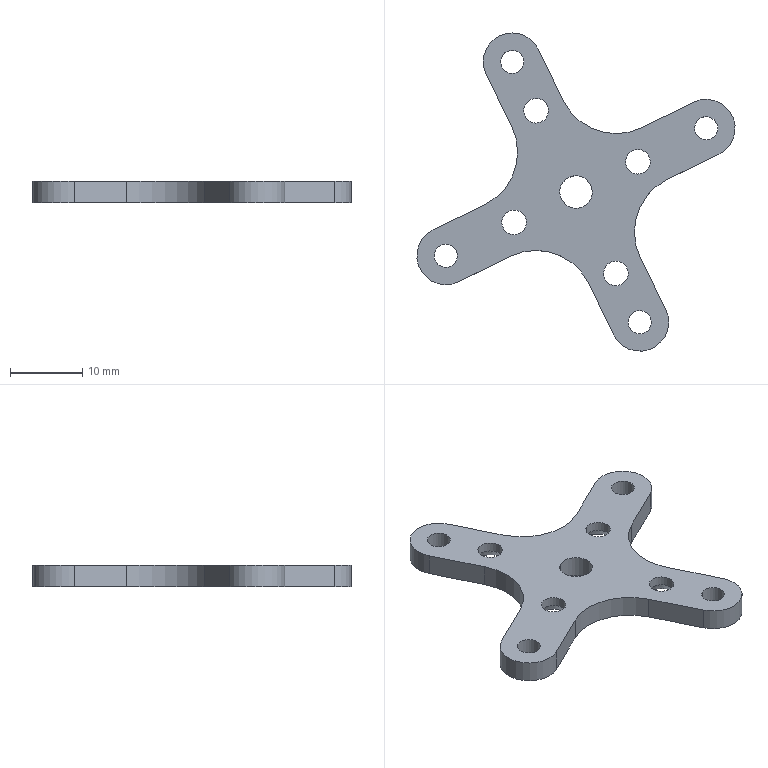Component | SolidWorks | BaseConnectionPart-1 | 1 solid | 45 faces | box 43.92 x 43.92 x 3 mm | volume 1875 mm3 | cylinder 27 | plane 10 | cone 8 | commonest cylinder face diameters 3.4 x8 3.2 x8 8 x5 16 x4 4.5 x2
build123d program:
from build123d import *

# Parameters (mm, degrees)
SKETCH1_R                                            = 1.6
BOSS_EXTRUDE1_DEPTH                                  = 3
CONICAL_COUNTERSUNK_HOLE_FOR_M6_HEXALOBU_D           = 3.4
CONICAL_COUNTERSUNK_HOLE_FOR_M6_HEXALOBU_DEPTH       = 8.5
CONICAL_COUNTERSUNK_HOLE_FOR_M6_HEXALOBU_CSINK_D     = 6.3
CONICAL_COUNTERSUNK_HOLE_FOR_M6_HEXALOBU_CSINK_ANGLE = 82
CONICAL_COUNTERSUNK_HOLE_FOR_M6_HEXALOBU_TIP         = 1.021
SKETCH4_R                                            = 2.25
CUT_EXTRUDE1_DEPTH                                   = 35.073


with BuildPart() as part:
    # Sketch1 → Boss-Extrude1 (new body)
    with BuildSketch(Plane.XY):
        with BuildLine():
            ThreePointArc((4, 20), (2.828, 22.828), (0, 24))
            ThreePointArc((0, 24), (-2.828, 22.828), (-4, 20))
            Line((-4, 20), (-4, 12))
            ThreePointArc((-4, 12), (-6.343, 6.343), (-12, 4))
            Line((-12, 4), (-20, 4))
            ThreePointArc((-20, 4), (-22.828, 2.828), (-24, 0))
            ThreePointArc((-24, 0), (-22.828, -2.828), (-20, -4))
            Line((-20, -4), (-12, -4))
            ThreePointArc((-12, -4), (-6.343, -6.343), (-4, -12))
            Line((-4, -12), (-4, -20))
            ThreePointArc((-4, -20), (-2.828, -22.828), (0, -24))
            ThreePointArc((0, -24), (2.828, -22.828), (4, -20))
            Line((4, -20), (4, -12))
            ThreePointArc((4, -12), (6.343, -6.343), (12, -4))
            Line((12, -4), (20, -4))
            ThreePointArc((20, -4), (22.828, -2.828), (24, 0))
            ThreePointArc((24, 0), (22.828, 2.828), (20, 4))
            Line((20, 4), (12, 4))
            ThreePointArc((12, 4), (6.343, 6.343), (4, 12))
            Line((4, 12), (4, 20))
        make_face()
        with Locations((0, 20)):
            Circle(SKETCH1_R, mode=Mode.SUBTRACT)
        with Locations((20, 0)):
            Circle(SKETCH1_R, mode=Mode.SUBTRACT)
        with Locations((0, -20)):
            Circle(SKETCH1_R, mode=Mode.SUBTRACT)
        with Locations((-20, 0)):
            Circle(SKETCH1_R, mode=Mode.SUBTRACT)
    extrude(amount=BOSS_EXTRUDE1_DEPTH)

    # Conical Countersunk Hole for M6 Hexalobu
    with Locations(Plane(origin=(0, 0, 0), x_dir=(-1, 0, 0), z_dir=(0, 0, -1))):
        with Locations((-12.5, 0), (0, 9.5), (12.5, 0), (0, -9.5)):
            CounterSinkHole(CONICAL_COUNTERSUNK_HOLE_FOR_M6_HEXALOBU_D / 2, CONICAL_COUNTERSUNK_HOLE_FOR_M6_HEXALOBU_CSINK_D / 2, depth=CONICAL_COUNTERSUNK_HOLE_FOR_M6_HEXALOBU_DEPTH, counter_sink_angle=CONICAL_COUNTERSUNK_HOLE_FOR_M6_HEXALOBU_CSINK_ANGLE)
            with Locations((0, 0, -(CONICAL_COUNTERSUNK_HOLE_FOR_M6_HEXALOBU_DEPTH + CONICAL_COUNTERSUNK_HOLE_FOR_M6_HEXALOBU_TIP / 2))):  # 118° drill point
                Cone(0, CONICAL_COUNTERSUNK_HOLE_FOR_M6_HEXALOBU_D / 2, CONICAL_COUNTERSUNK_HOLE_FOR_M6_HEXALOBU_TIP, mode=Mode.SUBTRACT)

    # Sketch4 → Cut-Extrude1 (cut, through all)
    with BuildSketch(Plane.XY.offset(3)):
        Circle(SKETCH4_R)
    extrude(amount=-CUT_EXTRUDE1_DEPTH, mode=Mode.SUBTRACT)


solid = part.part

# Placed as in the assembly
solid = solid.moved(Location((-218.606, 95.367, 1039.6), (0, 0, 116.091)))